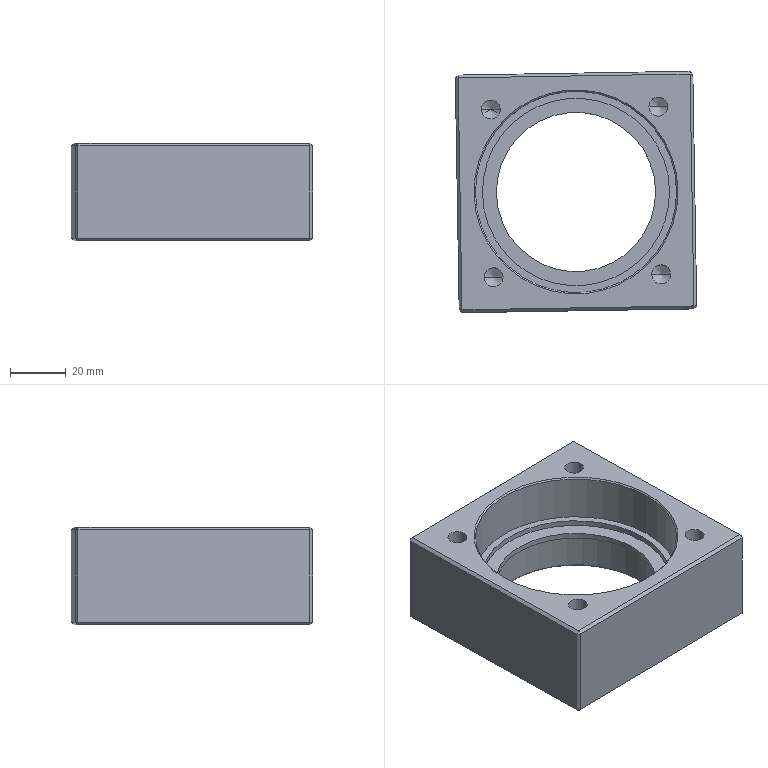Component | SolidWorks | 8TC-A17001-20-01BearingHousing-1 | 1 solid | 69 faces | volume 124536 mm3 | plane 29 | cylinder 22 | cone 18 | commonest cylinder face diameters 6.8 x8 5 x6 67 x2 62 x2 72 x2 57 x2 | material #45